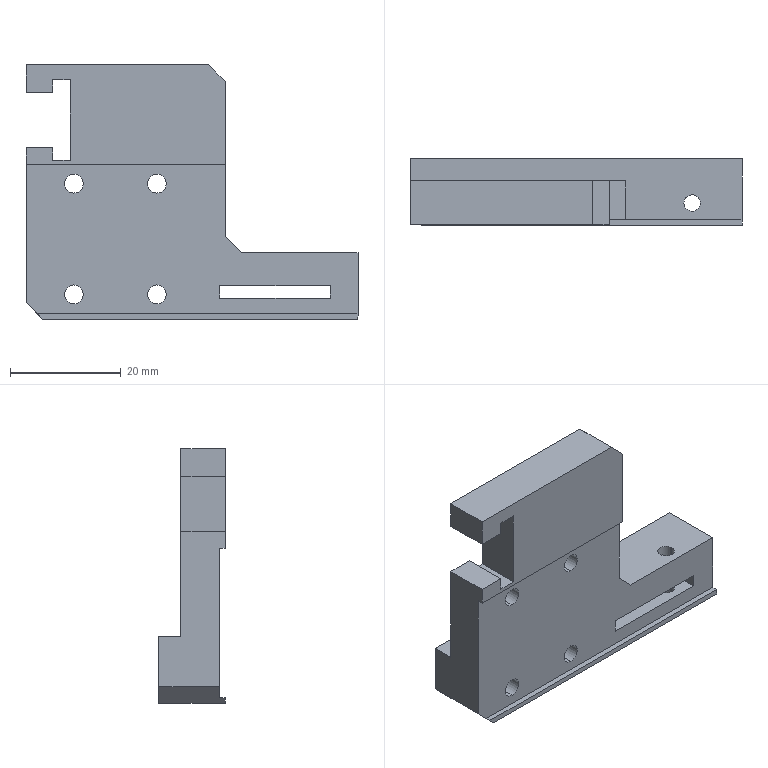Component | SolidWorks | 17268060-1 | 1 solid | 59 faces | box 60 x 12 x 46 mm | volume 14813 mm3 | plane 34 | cylinder 25 | commonest cylinder face diameters 6.5 x8 3.4 x8 3 x4 3.5 x3 2.5 x2 | material S136H FINISH:HRC50~52 degrees
build123d program:
from build123d import *

# Parameters (mm, degrees)
SKETCH1_W                                       = 180
SKETCH1_H                                       = 12
BOSS_EXTRUDE1_DEPTH                             = 12
SKETCH7_W                                       = 8
SKETCH7_H                                       = 6
CUT_EXTRUDE6_DEPTH                              = 181.798
SKETCH8_R                                       = 1.5
CUT_EXTRUDE7_DEPTH                              = 181.499
SKETCH9_W                                       = 44.5
SKETCH9_H                                       = 12
CUT_EXTRUDE8_DEPTH                              = 181.798
SIZE_MM_DOWEL_PIN_HOLE1_D                       = 3
SKETCH12_W                                      = 20
SKETCH12_H                                      = 2.3
CUT_EXTRUDE9_DEPTH                              = 181.798
SKETCH13_W                                      = 75.5
SKETCH13_H                                      = 12
CUT_EXTRUDE10_DEPTH                             = 181.798
SKETCH14_W                                      = 36
SKETCH14_H                                      = 8
BOSS_EXTRUDE2_DEPTH                             = 34
SKETCH15_W                                      = 27
SKETCH15_H                                      = 1
CUT_EXTRUDE11_DEPTH                             = 71
CUT_EXTRUDE12_DEPTH                             = 111.183
M3_HEX_SOCKET_HEAD_CAP_SCREW_CBORE1_D           = 3.4
M3_HEX_SOCKET_HEAD_CAP_SCREW_CBORE1_CBORE_D     = 6.5
M3_HEX_SOCKET_HEAD_CAP_SCREW_CBORE1_CBORE_DEPTH = 8.4
CHAMFER1_SIZE                                   = 3
SKETCH20_R                                      = 1.75
CUT_EXTRUDE13_DEPTH                             = 8
M3_TAPPED_HOLE1_REACH                           = 112.545
M3_TAPPED_HOLE1_BORE_R                          = 1.25


with BuildPart() as part:
    # Sketch1 → Boss-Extrude1 (new body)
    with BuildSketch(Plane.XY):
        with Locations((90, 6)):
            Rectangle(SKETCH1_W, SKETCH1_H)
    extrude(amount=BOSS_EXTRUDE1_DEPTH)

    # Sketch7 → Cut-Extrude6 (cut, through all)
    with BuildSketch(Plane.XY.offset(12)):
        with Locations((176, 9)):
            Rectangle(SKETCH7_W, SKETCH7_H)
    extrude(amount=-CUT_EXTRUDE6_DEPTH, mode=Mode.SUBTRACT)

    # Sketch8 → Cut-Extrude7 (cut, through all)
    with BuildSketch(Plane(origin=(0, 6, 0), x_dir=(1, 0, 0), z_dir=(0, 1, 0))):
        with Locations(Location((176, -6, 0), (0, 0, 180))):
            Circle(SKETCH8_R)
    extrude(amount=-CUT_EXTRUDE7_DEPTH, mode=Mode.SUBTRACT)

    # Sketch9 → Cut-Extrude8 (cut, through all)
    with BuildSketch(Plane.XZ):
        with Locations((22.25, 6)):
            Rectangle(SKETCH9_W, SKETCH9_H)
    extrude(amount=-CUT_EXTRUDE8_DEPTH, mode=Mode.SUBTRACT)

    # Size mm Dowel Pin Hole1 (through all)
    with Locations(Plane(origin=(0, 0, 0), x_dir=(-1, 0, 0), z_dir=(0, 0, -1))):
        with Locations((-53.5, 4)):
            Hole(SIZE_MM_DOWEL_PIN_HOLE1_D / 2)

    # Sketch12 → Cut-Extrude9 (cut, through all)
    with BuildSketch(Plane(origin=(0, 12, 0), x_dir=(1, 0, 0), z_dir=(0, 1, 0))):
        with Locations((59.5, -7.05)):
            Rectangle(SKETCH12_W, SKETCH12_H)
    extrude(amount=-CUT_EXTRUDE9_DEPTH, mode=Mode.SUBTRACT)

    # Sketch13 → Cut-Extrude10 (cut, through all)
    with BuildSketch(Plane(origin=(0, 0, 0), x_dir=(-1, 0, 0), z_dir=(0, 0, -1))):
        with Locations((-142.25, 6)):
            Rectangle(SKETCH13_W, SKETCH13_H)
    extrude(amount=-CUT_EXTRUDE10_DEPTH, mode=Mode.SUBTRACT)

    # Sketch14 → Boss-Extrude2 (add)
    with BuildSketch(Plane(origin=(0, 0, 0), x_dir=(-1, 0, 0), z_dir=(0, 0, -1))):
        with Locations((-86.5, 4)):
            Rectangle(SKETCH14_W, SKETCH14_H)
    extrude(amount=BOSS_EXTRUDE2_DEPTH)

    # Sketch15 → Cut-Extrude11 (cut, through all)
    with BuildSketch(Plane(origin=(104.5, 0, 0), x_dir=(0, 0, -1), z_dir=(1, 0, 0))):
        with Locations((2.5, 0.5)):
            Rectangle(SKETCH15_W, SKETCH15_H)
    extrude(amount=-CUT_EXTRUDE11_DEPTH, mode=Mode.SUBTRACT)

    # Sketch16 → Cut-Extrude12 (cut, through all)
    with BuildSketch(Plane(origin=(0, 8, 0), x_dir=(1, 0, 0), z_dir=(0, 1, 0))):
        Polygon((104.5, 29), (99.7, 29), (99.7, 31.3), (96.5, 31.3), (96.5, 16.7), (99.7, 16.7), (99.7, 19), (104.5, 19), align=None)
    extrude(amount=-CUT_EXTRUDE12_DEPTH, mode=Mode.SUBTRACT)

    # M3 Hex Socket Head Cap Screw CBORE1 (through all)
    with Locations(Plane(origin=(0, 12, 0), x_dir=(1, 0, 0), z_dir=(0, 1, 0))):
        with Locations((80.85, -7.5), (95.85, -7.5), (80.85, 12.5), (95.85, 12.5)):
            CounterBoreHole(M3_HEX_SOCKET_HEAD_CAP_SCREW_CBORE1_D / 2, M3_HEX_SOCKET_HEAD_CAP_SCREW_CBORE1_CBORE_D / 2, M3_HEX_SOCKET_HEAD_CAP_SCREW_CBORE1_CBORE_DEPTH)

    # Chamfer1
    chamfer1_edges = [part.edges().sort_by_distance(p)[0] for p in [
        (104.5, 6, 12),
        (68.5, 4, -34),
        (68.5, 4.5, 0),
    ]]
    chamfer(chamfer1_edges, length=CHAMFER1_SIZE)

    # Sketch20 → Cut-Extrude13 (cut)
    with BuildSketch(Plane(origin=(0, 12, 0), x_dir=(1, 0, 0), z_dir=(0, 1, 0))):
        with Locations((62.5, -7.05)):
            Circle(SKETCH20_R)
    extrude(amount=-CUT_EXTRUDE13_DEPTH, mode=Mode.SUBTRACT)

    # M3 Tapped Hole1 bore → M3 Tapped Hole1 (cut, up to next)
    with BuildSketch(Plane(origin=(0, 12, 0), x_dir=(1, 0, 0), z_dir=(0, 1, 0)), mode=Mode.PRIVATE) as m3_tapped_hole1_sk1:
        with Locations((53.5, -2.95)):
            Circle(M3_TAPPED_HOLE1_BORE_R)
    m3_tapped_hole1_tool1 = extrude(m3_tapped_hole1_sk1.sketch, amount=-M3_TAPPED_HOLE1_REACH, mode=Mode.PRIVATE) & part.part
    add(m3_tapped_hole1_tool1.solids().sort_by_distance((53.5, 12, 2.95))[0], mode=Mode.SUBTRACT)


solid = part.part

# Placed as in the assembly
solid = solid.moved(Location((111, -31.579, -2.5), (-180, 0, 180)))